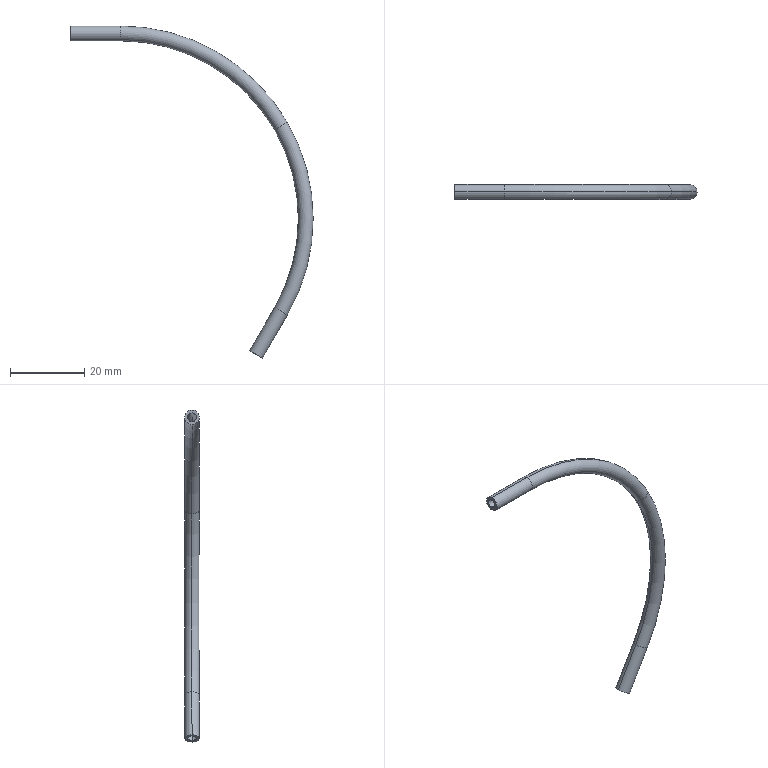Component | SolidWorks | WaterPipe1-2 | 1 solid | 18 faces | box 65.4 x 4 x 89.6 mm | volume 1058 mm3 | torus 8 | cylinder 8 | plane 2 | commonest cylinder face diameters 2.4 x4 4 x4
build123d program:
from build123d import *

# Parameters (mm, degrees)
SCAN_THIN_FEATURE1_PROFILE_R   = 2
SCAN_THIN_FEATURE1_PROFILE_R_2 = 1.2


with BuildPart() as part:
    # Scan-Thin Feature1: sweep along a path in Sketch1
    with BuildLine(Plane(origin=(0, 0, 0), x_dir=(1, 0, 0), z_dir=(0, 1, 0))) as scan_thin_feature1_path:
        Line((-50, 86.603), (-43.301, 75))
        ThreePointArc((-43.301, 75), (0, 50), (43.301, 75))
        Line((43.301, 75), (50, 86.603))
    # Scan-Thin Feature1 profile (on start of the path) → Scan-Thin Feature1 (sweep)
    with BuildSketch(Plane(origin=(-50, 0, -86.603), x_dir=(0.866, 0, -0.5), z_dir=(0.5, 0, 0.866))):
        Circle(SCAN_THIN_FEATURE1_PROFILE_R)
        Circle(SCAN_THIN_FEATURE1_PROFILE_R_2, mode=Mode.SUBTRACT)
    sweep(path=scan_thin_feature1_path.line)


solid = part.part

# Placed as in the assembly
solid = solid.moved(Location((104.985, 33.561, 224.066), (0, 60, 0)))
STEP:
#1=CARTESIAN_POINT('',(2.388,1.321,5.892));
#2=VERTEX_POINT('',#1);
#3=CARTESIAN_POINT('',(2.469,1.321,5.845));
#4=VERTEX_POINT('',#3);
#5=CARTESIAN_POINT('',(2.429,1.321,5.869));
#6=DIRECTION('',(-0.5,-0.,-0.866));
#7=DIRECTION('',(-0.866,0.,0.5));
#8=AXIS2_PLACEMENT_3D('',#5,#6,#7);
#9=CIRCLE('',#8,0.04724);
#10=EDGE_CURVE('',#2,#4,#9,.T.);
#11=ORIENTED_EDGE('',*,*,#10,.T.);
#12=CARTESIAN_POINT('',(2.469,1.321,7.861));
#13=VERTEX_POINT('',#12);
#14=CARTESIAN_POINT('',(0.7237,1.321,6.853));
#15=DIRECTION('',(0.,-1.,-0.));
#16=DIRECTION('',(1.,0.,0.));
#17=AXIS2_PLACEMENT_3D('',#14,#15,#16);
#18=CIRCLE('',#17,2.016);
#19=EDGE_CURVE('',#4,#13,#18,.T.);
#20=ORIENTED_EDGE('',*,*,#19,.T.);
#21=CARTESIAN_POINT('',(2.388,1.321,7.814));
#22=VERTEX_POINT('',#21);
#23=CARTESIAN_POINT('',(2.429,1.321,7.837));
#24=DIRECTION('',(0.5,0.,-0.866));
#25=DIRECTION('',(-0.866,0.,-0.5));
#26=AXIS2_PLACEMENT_3D('',#23,#24,#25);
#27=CIRCLE('',#26,0.04724);
#28=EDGE_CURVE('',#22,#13,#27,.T.);
#29=ORIENTED_EDGE('',*,*,#28,.F.);
#30=CARTESIAN_POINT('',(0.7237,1.321,6.853));
#31=DIRECTION('',(0.,-1.,-0.));
#32=DIRECTION('',(1.,0.,0.));
#33=AXIS2_PLACEMENT_3D('',#30,#31,#32);
#34=CIRCLE('',#33,1.921);
#35=EDGE_CURVE('',#2,#22,#34,.T.);
#36=ORIENTED_EDGE('',*,*,#35,.F.);
#37=EDGE_LOOP('',(#11,#20,#29,#36));
#38=FACE_OUTER_BOUND('',#37,.T.);
#39=CARTESIAN_POINT('',(0.7237,1.321,6.853));
#40=DIRECTION('',(0.,-1.,-0.));
#41=DIRECTION('',(0.866,0.,0.5));
#42=AXIS2_PLACEMENT_3D('',#39,#40,#41);
#43=TOROIDAL_SURFACE('',#42,1.969,0.04724);
#44=ADVANCED_FACE('',(#38),#43,.F.);
#45=CARTESIAN_POINT('',(2.497,1.321,7.877));
#46=VERTEX_POINT('',#45);
#47=CARTESIAN_POINT('',(2.36,1.321,7.798));
#48=VERTEX_POINT('',#47);
#49=CARTESIAN_POINT('',(2.429,1.321,7.837));
#50=DIRECTION('',(0.5,0.,-0.866));
#51=DIRECTION('',(-0.866,0.,-0.5));
#52=AXIS2_PLACEMENT_3D('',#49,#50,#51);
#53=CIRCLE('',#52,0.07874);
#54=EDGE_CURVE('',#46,#48,#53,.T.);
#55=ORIENTED_EDGE('',*,*,#54,.F.);
#56=CARTESIAN_POINT('',(0.7237,1.321,8.9));
#57=VERTEX_POINT('',#56);
#58=CARTESIAN_POINT('',(0.7237,1.321,6.853));
#59=DIRECTION('',(0.,-1.,-0.));
#60=DIRECTION('',(1.,0.,0.));
#61=AXIS2_PLACEMENT_3D('',#58,#59,#60);
#62=CIRCLE('',#61,2.047);
#63=EDGE_CURVE('',#46,#57,#62,.T.);
#64=ORIENTED_EDGE('',*,*,#63,.T.);
#65=CARTESIAN_POINT('',(0.7237,1.321,8.743));
#66=VERTEX_POINT('',#65);
#67=CARTESIAN_POINT('',(0.7237,1.321,8.822));
#68=DIRECTION('',(1.,0.,-0.));
#69=DIRECTION('',(0.,0.,1.));
#70=AXIS2_PLACEMENT_3D('',#67,#68,#69);
#71=CIRCLE('',#70,0.07874);
#72=EDGE_CURVE('',#57,#66,#71,.T.);
#73=ORIENTED_EDGE('',*,*,#72,.T.);
#74=CARTESIAN_POINT('',(0.7237,1.321,6.853));
#75=DIRECTION('',(0.,-1.,-0.));
#76=DIRECTION('',(1.,0.,0.));
#77=AXIS2_PLACEMENT_3D('',#74,#75,#76);
#78=CIRCLE('',#77,1.89);
#79=EDGE_CURVE('',#48,#66,#78,.T.);
#80=ORIENTED_EDGE('',*,*,#79,.F.);
#81=EDGE_LOOP('',(#55,#64,#73,#80));
#82=FACE_OUTER_BOUND('',#81,.T.);
#83=CARTESIAN_POINT('',(0.7237,1.321,6.853));
#84=DIRECTION('',(0.,-1.,-0.));
#85=DIRECTION('',(0.866,0.,0.5));
#86=AXIS2_PLACEMENT_3D('',#83,#84,#85);
#87=TOROIDAL_SURFACE('',#86,1.969,0.07874);
#88=ADVANCED_FACE('',(#82),#87,.T.);
#89=CARTESIAN_POINT('',(2.497,1.321,5.829));
#90=VERTEX_POINT('',#89);
#91=CARTESIAN_POINT('',(2.36,1.321,5.908));
#92=VERTEX_POINT('',#91);
#93=CARTESIAN_POINT('',(2.429,1.321,5.869));
#94=DIRECTION('',(-0.5,-0.,-0.866));
#95=DIRECTION('',(0.866,0.,-0.5));
#96=AXIS2_PLACEMENT_3D('',#93,#94,#95);
#97=CIRCLE('',#96,0.07874);
#98=EDGE_CURVE('',#90,#92,#97,.T.);
#99=ORIENTED_EDGE('',*,*,#98,.F.);
#100=CARTESIAN_POINT('',(0.7237,1.321,6.853));
#101=DIRECTION('',(0.,-1.,-0.));
#102=DIRECTION('',(1.,0.,0.));
#103=AXIS2_PLACEMENT_3D('',#100,#101,#102);
#104=CIRCLE('',#103,2.047);
#105=EDGE_CURVE('',#90,#46,#104,.T.);
#106=ORIENTED_EDGE('',*,*,#105,.T.);
#107=ORIENTED_EDGE('',*,*,#54,.T.);
#108=CARTESIAN_POINT('',(0.7237,1.321,6.853));
#109=DIRECTION('',(0.,-1.,-0.));
#110=DIRECTION('',(1.,0.,0.));
#111=AXIS2_PLACEMENT_3D('',#108,#109,#110);
#112=CIRCLE('',#111,1.89);
#113=EDGE_CURVE('',#92,#48,#112,.T.);
#114=ORIENTED_EDGE('',*,*,#113,.F.);
#115=EDGE_LOOP('',(#99,#106,#107,#114));
#116=FACE_OUTER_BOUND('',#115,.T.);
#117=CARTESIAN_POINT('',(0.7237,1.321,6.853));
#118=DIRECTION('',(0.,-1.,-0.));
#119=DIRECTION('',(0.866,0.,0.5));
#120=AXIS2_PLACEMENT_3D('',#117,#118,#119);
#121=TOROIDAL_SURFACE('',#120,1.969,0.07874);
#122=ADVANCED_FACE('',(#116),#121,.T.);
#123=ORIENTED_EDGE('',*,*,#28,.T.);
#124=CARTESIAN_POINT('',(0.7237,1.321,8.869));
#125=VERTEX_POINT('',#124);
#126=CARTESIAN_POINT('',(0.7237,1.321,6.853));
#127=DIRECTION('',(0.,-1.,-0.));
#128=DIRECTION('',(1.,0.,0.));
#129=AXIS2_PLACEMENT_3D('',#126,#127,#128);
#130=CIRCLE('',#129,2.016);
#131=EDGE_CURVE('',#13,#125,#130,.T.);
#132=ORIENTED_EDGE('',*,*,#131,.T.);
#133=CARTESIAN_POINT('',(0.7237,1.321,8.774));
#134=VERTEX_POINT('',#133);
#135=CARTESIAN_POINT('',(0.7237,1.321,8.822));
#136=DIRECTION('',(1.,0.,0.));
#137=DIRECTION('',(-0.,0.,1.));
#138=AXIS2_PLACEMENT_3D('',#135,#136,#137);
#139=CIRCLE('',#138,0.04724);
#140=EDGE_CURVE('',#134,#125,#139,.T.);
#141=ORIENTED_EDGE('',*,*,#140,.F.);
#142=CARTESIAN_POINT('',(0.7237,1.321,6.853));
#143=DIRECTION('',(0.,-1.,-0.));
#144=DIRECTION('',(1.,0.,0.));
#145=AXIS2_PLACEMENT_3D('',#142,#143,#144);
#146=CIRCLE('',#145,1.921);
#147=EDGE_CURVE('',#22,#134,#146,.T.);
#148=ORIENTED_EDGE('',*,*,#147,.F.);
#149=EDGE_LOOP('',(#123,#132,#141,#148));
#150=FACE_OUTER_BOUND('',#149,.T.);
#151=CARTESIAN_POINT('',(0.7237,1.321,6.853));
#152=DIRECTION('',(0.,-1.,-0.));
#153=DIRECTION('',(0.866,0.,0.5));
#154=AXIS2_PLACEMENT_3D('',#151,#152,#153);
#155=TOROIDAL_SURFACE('',#154,1.969,0.04724);
#156=ADVANCED_FACE('',(#150),#155,.F.);
#157=ORIENTED_EDGE('',*,*,#140,.T.);
#158=CARTESIAN_POINT('',(0.1963,1.321,8.869));
#159=VERTEX_POINT('',#158);
#160=CARTESIAN_POINT('',(0.7237,1.321,8.869));
#161=DIRECTION('',(-1.,-0.,0.));
#162=VECTOR('',#161,39.37);
#163=LINE('',#160,#162);
#164=EDGE_CURVE('',#125,#159,#163,.T.);
#165=ORIENTED_EDGE('',*,*,#164,.T.);
#166=CARTESIAN_POINT('',(0.1963,1.321,8.774));
#167=VERTEX_POINT('',#166);
#168=CARTESIAN_POINT('',(0.1963,1.321,8.822));
#169=DIRECTION('',(1.,0.,-0.));
#170=DIRECTION('',(0.,0.,1.));
#171=AXIS2_PLACEMENT_3D('',#168,#169,#170);
#172=CIRCLE('',#171,0.04724);
#173=EDGE_CURVE('',#167,#159,#172,.T.);
#174=ORIENTED_EDGE('',*,*,#173,.F.);
#175=CARTESIAN_POINT('',(0.7237,1.321,8.774));
#176=DIRECTION('',(-1.,-0.,0.));
#177=VECTOR('',#176,39.37);
#178=LINE('',#175,#177);
#179=EDGE_CURVE('',#134,#167,#178,.T.);
#180=ORIENTED_EDGE('',*,*,#179,.F.);
#181=EDGE_LOOP('',(#157,#165,#174,#180));
#182=FACE_OUTER_BOUND('',#181,.T.);
#183=CARTESIAN_POINT('',(0.7237,1.321,8.822));
#184=DIRECTION('',(-1.,-0.,0.));
#185=DIRECTION('',(0.,0.,-1.));
#186=AXIS2_PLACEMENT_3D('',#183,#184,#185);
#187=CYLINDRICAL_SURFACE('',#186,0.04724);
#188=ADVANCED_FACE('',(#182),#187,.F.);
#189=ORIENTED_EDGE('',*,*,#131,.F.);
#190=CARTESIAN_POINT('',(2.429,1.321,7.837));
#191=DIRECTION('',(0.5,0.,-0.866));
#192=DIRECTION('',(-0.866,0.,-0.5));
#193=AXIS2_PLACEMENT_3D('',#190,#191,#192);
#194=CIRCLE('',#193,0.04724);
#195=EDGE_CURVE('',#13,#22,#194,.T.);
#196=ORIENTED_EDGE('',*,*,#195,.T.);
#197=ORIENTED_EDGE('',*,*,#147,.T.);
#198=CARTESIAN_POINT('',(0.7237,1.321,8.822));
#199=DIRECTION('',(1.,0.,0.));
#200=DIRECTION('',(-0.,0.,1.));
#201=AXIS2_PLACEMENT_3D('',#198,#199,#200);
#202=CIRCLE('',#201,0.04724);
#203=EDGE_CURVE('',#125,#134,#202,.T.);
#204=ORIENTED_EDGE('',*,*,#203,.F.);
#205=EDGE_LOOP('',(#189,#196,#197,#204));
#206=FACE_OUTER_BOUND('',#205,.T.);
#207=CARTESIAN_POINT('',(0.7237,1.321,6.853));
#208=DIRECTION('',(0.,-1.,-0.));
#209=DIRECTION('',(0.866,0.,0.5));
#210=AXIS2_PLACEMENT_3D('',#207,#208,#209);
#211=TOROIDAL_SURFACE('',#210,1.969,0.04724);
#212=ADVANCED_FACE('',(#206),#211,.F.);
#213=CARTESIAN_POINT('',(2.124,1.321,5.436));
#214=VERTEX_POINT('',#213);
#215=CARTESIAN_POINT('',(2.206,1.321,5.388));
#216=VERTEX_POINT('',#215);
#217=CARTESIAN_POINT('',(2.165,1.321,5.412));
#218=DIRECTION('',(-0.5,-0.,-0.866));
#219=DIRECTION('',(0.866,0.,-0.5));
#220=AXIS2_PLACEMENT_3D('',#217,#218,#219);
#221=CIRCLE('',#220,0.04724);
#222=EDGE_CURVE('',#214,#216,#221,.T.);
#223=ORIENTED_EDGE('',*,*,#222,.T.);
#224=CARTESIAN_POINT('',(2.206,1.321,5.388));
#225=DIRECTION('',(0.5,0.,0.866));
#226=VECTOR('',#225,39.37);
#227=LINE('',#224,#226);
#228=EDGE_CURVE('',#216,#4,#227,.T.);
#229=ORIENTED_EDGE('',*,*,#228,.T.);
#230=ORIENTED_EDGE('',*,*,#10,.F.);
#231=CARTESIAN_POINT('',(2.124,1.321,5.436));
#232=DIRECTION('',(0.5,0.,0.866));
#233=VECTOR('',#232,39.37);
#234=LINE('',#231,#233);
#235=EDGE_CURVE('',#214,#2,#234,.T.);
#236=ORIENTED_EDGE('',*,*,#235,.F.);
#237=EDGE_LOOP('',(#223,#229,#230,#236));
#238=FACE_OUTER_BOUND('',#237,.T.);
#239=CARTESIAN_POINT('',(2.165,1.321,5.412));
#240=DIRECTION('',(0.5,0.,0.866));
#241=DIRECTION('',(-0.866,0.,0.5));
#242=AXIS2_PLACEMENT_3D('',#239,#240,#241);
#243=CYLINDRICAL_SURFACE('',#242,0.04724);
#244=ADVANCED_FACE('',(#238),#243,.F.);
#245=ORIENTED_EDGE('',*,*,#72,.F.);
#246=CARTESIAN_POINT('',(0.1963,1.321,8.9));
#247=VERTEX_POINT('',#246);
#248=CARTESIAN_POINT('',(0.7237,1.321,8.9));
#249=DIRECTION('',(-1.,-0.,0.));
#250=VECTOR('',#249,39.37);
#251=LINE('',#248,#250);
#252=EDGE_CURVE('',#57,#247,#251,.T.);
#253=ORIENTED_EDGE('',*,*,#252,.T.);
#254=CARTESIAN_POINT('',(0.1963,1.321,8.743));
#255=VERTEX_POINT('',#254);
#256=CARTESIAN_POINT('',(0.1963,1.321,8.822));
#257=DIRECTION('',(1.,0.,-0.));
#258=DIRECTION('',(0.,0.,1.));
#259=AXIS2_PLACEMENT_3D('',#256,#257,#258);
#260=CIRCLE('',#259,0.07874);
#261=EDGE_CURVE('',#247,#255,#260,.T.);
#262=ORIENTED_EDGE('',*,*,#261,.T.);
#263=CARTESIAN_POINT('',(0.7237,1.321,8.743));
#264=DIRECTION('',(-1.,-0.,0.));
#265=VECTOR('',#264,39.37);
#266=LINE('',#263,#265);
#267=EDGE_CURVE('',#66,#255,#266,.T.);
#268=ORIENTED_EDGE('',*,*,#267,.F.);
#269=EDGE_LOOP('',(#245,#253,#262,#268));
#270=FACE_OUTER_BOUND('',#269,.T.);
#271=CARTESIAN_POINT('',(0.7237,1.321,8.822));
#272=DIRECTION('',(-1.,-0.,0.));
#273=DIRECTION('',(0.,0.,-1.));
#274=AXIS2_PLACEMENT_3D('',#271,#272,#273);
#275=CYLINDRICAL_SURFACE('',#274,0.07874);
#276=ADVANCED_FACE('',(#270),#275,.T.);
#277=ORIENTED_EDGE('',*,*,#105,.F.);
#278=CARTESIAN_POINT('',(2.429,1.321,5.869));
#279=DIRECTION('',(-0.5,-0.,-0.866));
#280=DIRECTION('',(0.866,0.,-0.5));
#281=AXIS2_PLACEMENT_3D('',#278,#279,#280);
#282=CIRCLE('',#281,0.07874);
#283=EDGE_CURVE('',#92,#90,#282,.T.);
#284=ORIENTED_EDGE('',*,*,#283,.F.);
#285=ORIENTED_EDGE('',*,*,#113,.T.);
#286=CARTESIAN_POINT('',(2.429,1.321,7.837));
#287=DIRECTION('',(0.5,0.,-0.866));
#288=DIRECTION('',(-0.866,0.,-0.5));
#289=AXIS2_PLACEMENT_3D('',#286,#287,#288);
#290=CIRCLE('',#289,0.07874);
#291=EDGE_CURVE('',#48,#46,#290,.T.);
#292=ORIENTED_EDGE('',*,*,#291,.T.);
#293=EDGE_LOOP('',(#277,#284,#285,#292));
#294=FACE_OUTER_BOUND('',#293,.T.);
#295=CARTESIAN_POINT('',(0.7237,1.321,6.853));
#296=DIRECTION('',(0.,-1.,-0.));
#297=DIRECTION('',(0.866,0.,0.5));
#298=AXIS2_PLACEMENT_3D('',#295,#296,#297);
#299=TOROIDAL_SURFACE('',#298,1.969,0.07874);
#300=ADVANCED_FACE('',(#294),#299,.T.);
#301=CARTESIAN_POINT('',(2.233,1.321,5.373));
#302=VERTEX_POINT('',#301);
#303=CARTESIAN_POINT('',(2.097,1.321,5.451));
#304=VERTEX_POINT('',#303);
#305=CARTESIAN_POINT('',(2.165,1.321,5.412));
#306=DIRECTION('',(-0.5,-0.,-0.866));
#307=DIRECTION('',(0.866,0.,-0.5));
#308=AXIS2_PLACEMENT_3D('',#305,#306,#307);
#309=CIRCLE('',#308,0.07874);
#310=EDGE_CURVE('',#302,#304,#309,.T.);
#311=ORIENTED_EDGE('',*,*,#310,.F.);
#312=CARTESIAN_POINT('',(2.233,1.321,5.373));
#313=DIRECTION('',(0.5,0.,0.866));
#314=VECTOR('',#313,39.37);
#315=LINE('',#312,#314);
#316=EDGE_CURVE('',#302,#90,#315,.T.);
#317=ORIENTED_EDGE('',*,*,#316,.T.);
#318=ORIENTED_EDGE('',*,*,#98,.T.);
#319=CARTESIAN_POINT('',(2.097,1.321,5.451));
#320=DIRECTION('',(0.5,0.,0.866));
#321=VECTOR('',#320,39.37);
#322=LINE('',#319,#321);
#323=EDGE_CURVE('',#304,#92,#322,.T.);
#324=ORIENTED_EDGE('',*,*,#323,.F.);
#325=EDGE_LOOP('',(#311,#317,#318,#324));
#326=FACE_OUTER_BOUND('',#325,.T.);
#327=CARTESIAN_POINT('',(2.165,1.321,5.412));
#328=DIRECTION('',(0.5,0.,0.866));
#329=DIRECTION('',(-0.866,0.,0.5));
#330=AXIS2_PLACEMENT_3D('',#327,#328,#329);
#331=CYLINDRICAL_SURFACE('',#330,0.07874);
#332=ADVANCED_FACE('',(#326),#331,.T.);
#333=ORIENTED_EDGE('',*,*,#252,.F.);
#334=CARTESIAN_POINT('',(0.7237,1.321,8.822));
#335=DIRECTION('',(1.,0.,-0.));
#336=DIRECTION('',(0.,0.,1.));
#337=AXIS2_PLACEMENT_3D('',#334,#335,#336);
#338=CIRCLE('',#337,0.07874);
#339=EDGE_CURVE('',#66,#57,#338,.T.);
#340=ORIENTED_EDGE('',*,*,#339,.F.);
#341=ORIENTED_EDGE('',*,*,#267,.T.);
#342=CARTESIAN_POINT('',(0.1963,1.321,8.822));
#343=DIRECTION('',(1.,0.,-0.));
#344=DIRECTION('',(0.,0.,1.));
#345=AXIS2_PLACEMENT_3D('',#342,#343,#344);
#346=CIRCLE('',#345,0.07874);
#347=EDGE_CURVE('',#255,#247,#346,.T.);
#348=ORIENTED_EDGE('',*,*,#347,.T.);
#349=EDGE_LOOP('',(#333,#340,#341,#348));
#350=FACE_OUTER_BOUND('',#349,.T.);
#351=CARTESIAN_POINT('',(0.7237,1.321,8.822));
#352=DIRECTION('',(-1.,-0.,0.));
#353=DIRECTION('',(0.,0.,-1.));
#354=AXIS2_PLACEMENT_3D('',#351,#352,#353);
#355=CYLINDRICAL_SURFACE('',#354,0.07874);
#356=ADVANCED_FACE('',(#350),#355,.T.);
#357=ORIENTED_EDGE('',*,*,#63,.F.);
#358=ORIENTED_EDGE('',*,*,#291,.F.);
#359=ORIENTED_EDGE('',*,*,#79,.T.);
#360=ORIENTED_EDGE('',*,*,#339,.T.);
#361=EDGE_LOOP('',(#357,#358,#359,#360));
#362=FACE_OUTER_BOUND('',#361,.T.);
#363=CARTESIAN_POINT('',(0.7237,1.321,6.853));
#364=DIRECTION('',(0.,-1.,-0.));
#365=DIRECTION('',(0.866,0.,0.5));
#366=AXIS2_PLACEMENT_3D('',#363,#364,#365);
#367=TOROIDAL_SURFACE('',#366,1.969,0.07874);
#368=ADVANCED_FACE('',(#362),#367,.T.);
#369=ORIENTED_EDGE('',*,*,#316,.F.);
#370=CARTESIAN_POINT('',(2.165,1.321,5.412));
#371=DIRECTION('',(-0.5,-0.,-0.866));
#372=DIRECTION('',(0.866,0.,-0.5));
#373=AXIS2_PLACEMENT_3D('',#370,#371,#372);
#374=CIRCLE('',#373,0.07874);
#375=EDGE_CURVE('',#304,#302,#374,.T.);
#376=ORIENTED_EDGE('',*,*,#375,.F.);
#377=ORIENTED_EDGE('',*,*,#323,.T.);
#378=ORIENTED_EDGE('',*,*,#283,.T.);
#379=EDGE_LOOP('',(#369,#376,#377,#378));
#380=FACE_OUTER_BOUND('',#379,.T.);
#381=CARTESIAN_POINT('',(2.165,1.321,5.412));
#382=DIRECTION('',(0.5,0.,0.866));
#383=DIRECTION('',(-0.866,0.,0.5));
#384=AXIS2_PLACEMENT_3D('',#381,#382,#383);
#385=CYLINDRICAL_SURFACE('',#384,0.07874);
#386=ADVANCED_FACE('',(#380),#385,.T.);
#387=ORIENTED_EDGE('',*,*,#173,.T.);
#388=CARTESIAN_POINT('',(0.1963,1.321,8.822));
#389=DIRECTION('',(1.,0.,-0.));
#390=DIRECTION('',(0.,0.,1.));
#391=AXIS2_PLACEMENT_3D('',#388,#389,#390);
#392=CIRCLE('',#391,0.04724);
#393=EDGE_CURVE('',#159,#167,#392,.T.);
#394=ORIENTED_EDGE('',*,*,#393,.T.);
#395=EDGE_LOOP('',(#387,#394));
#396=FACE_BOUND('',#395,.T.);
#397=ORIENTED_EDGE('',*,*,#347,.F.);
#398=ORIENTED_EDGE('',*,*,#261,.F.);
#399=EDGE_LOOP('',(#397,#398));
#400=FACE_OUTER_BOUND('',#399,.T.);
#401=CARTESIAN_POINT('',(0.1963,1.321,8.822));
#402=DIRECTION('',(1.,0.,-0.));
#403=DIRECTION('',(0.,0.,1.));
#404=AXIS2_PLACEMENT_3D('',#401,#402,#403);
#405=PLANE('',#404);
#406=ADVANCED_FACE('',(#396,#400),#405,.F.);
#407=ORIENTED_EDGE('',*,*,#222,.F.);
#408=CARTESIAN_POINT('',(2.165,1.321,5.412));
#409=DIRECTION('',(-0.5,-0.,-0.866));
#410=DIRECTION('',(0.866,0.,-0.5));
#411=AXIS2_PLACEMENT_3D('',#408,#409,#410);
#412=CIRCLE('',#411,0.04724);
#413=EDGE_CURVE('',#216,#214,#412,.T.);
#414=ORIENTED_EDGE('',*,*,#413,.F.);
#415=EDGE_LOOP('',(#407,#414));
#416=FACE_BOUND('',#415,.T.);
#417=ORIENTED_EDGE('',*,*,#375,.T.);
#418=ORIENTED_EDGE('',*,*,#310,.T.);
#419=EDGE_LOOP('',(#417,#418));
#420=FACE_OUTER_BOUND('',#419,.T.);
#421=CARTESIAN_POINT('',(2.165,1.321,5.412));
#422=DIRECTION('',(-0.5,-0.,-0.866));
#423=DIRECTION('',(0.866,0.,-0.5));
#424=AXIS2_PLACEMENT_3D('',#421,#422,#423);
#425=PLANE('',#424);
#426=ADVANCED_FACE('',(#416,#420),#425,.T.);
#427=ORIENTED_EDGE('',*,*,#164,.F.);
#428=ORIENTED_EDGE('',*,*,#203,.T.);
#429=ORIENTED_EDGE('',*,*,#179,.T.);
#430=ORIENTED_EDGE('',*,*,#393,.F.);
#431=EDGE_LOOP('',(#427,#428,#429,#430));
#432=FACE_OUTER_BOUND('',#431,.T.);
#433=CARTESIAN_POINT('',(0.7237,1.321,8.822));
#434=DIRECTION('',(-1.,-0.,0.));
#435=DIRECTION('',(0.,0.,-1.));
#436=AXIS2_PLACEMENT_3D('',#433,#434,#435);
#437=CYLINDRICAL_SURFACE('',#436,0.04724);
#438=ADVANCED_FACE('',(#432),#437,.F.);
#439=ORIENTED_EDGE('',*,*,#19,.F.);
#440=CARTESIAN_POINT('',(2.429,1.321,5.869));
#441=DIRECTION('',(-0.5,-0.,-0.866));
#442=DIRECTION('',(-0.866,0.,0.5));
#443=AXIS2_PLACEMENT_3D('',#440,#441,#442);
#444=CIRCLE('',#443,0.04724);
#445=EDGE_CURVE('',#4,#2,#444,.T.);
#446=ORIENTED_EDGE('',*,*,#445,.T.);
#447=ORIENTED_EDGE('',*,*,#35,.T.);
#448=ORIENTED_EDGE('',*,*,#195,.F.);
#449=EDGE_LOOP('',(#439,#446,#447,#448));
#450=FACE_OUTER_BOUND('',#449,.T.);
#451=CARTESIAN_POINT('',(0.7237,1.321,6.853));
#452=DIRECTION('',(0.,-1.,-0.));
#453=DIRECTION('',(0.866,0.,0.5));
#454=AXIS2_PLACEMENT_3D('',#451,#452,#453);
#455=TOROIDAL_SURFACE('',#454,1.969,0.04724);
#456=ADVANCED_FACE('',(#450),#455,.F.);
#457=ORIENTED_EDGE('',*,*,#228,.F.);
#458=ORIENTED_EDGE('',*,*,#413,.T.);
#459=ORIENTED_EDGE('',*,*,#235,.T.);
#460=ORIENTED_EDGE('',*,*,#445,.F.);
#461=EDGE_LOOP('',(#457,#458,#459,#460));
#462=FACE_OUTER_BOUND('',#461,.T.);
#463=CARTESIAN_POINT('',(2.165,1.321,5.412));
#464=DIRECTION('',(0.5,0.,0.866));
#465=DIRECTION('',(-0.866,0.,0.5));
#466=AXIS2_PLACEMENT_3D('',#463,#464,#465);
#467=CYLINDRICAL_SURFACE('',#466,0.04724);
#468=ADVANCED_FACE('',(#462),#467,.F.);
#469=CLOSED_SHELL('',(#44,#88,#122,#156,#188,#212,#244,#276,#300,#332,#356,#368,#386,#406,#426,#438,#456,#468));
#470=MANIFOLD_SOLID_BREP('',#469);
#471=CARTESIAN_POINT('',(0.,0.,0.));
#472=DIRECTION('',(0.,0.,1.));
#473=DIRECTION('',(1.,0.,0.));
#474=AXIS2_PLACEMENT_3D('',#471,#472,#473);
#475=(LENGTH_UNIT()NAMED_UNIT(*)SI_UNIT($,.METRE.));
#476=LENGTH_MEASURE_WITH_UNIT(LENGTH_MEASURE(0.0254),#475);
#477=DIMENSIONAL_EXPONENTS(1.,0.,0.,0.,0.,0.,0.);
#478=(CONVERSION_BASED_UNIT('',#476)LENGTH_UNIT()NAMED_UNIT(#477));
#479=UNCERTAINTY_MEASURE_WITH_UNIT(LENGTH_MEASURE(0.00001),#478,'','');
#480=(NAMED_UNIT(*)PLANE_ANGLE_UNIT()SI_UNIT($,.RADIAN.));
#481=(NAMED_UNIT(*)SI_UNIT($,.STERADIAN.)SOLID_ANGLE_UNIT());
#482=(GEOMETRIC_REPRESENTATION_CONTEXT(3)GLOBAL_UNCERTAINTY_ASSIGNED_CONTEXT((#479))GLOBAL_UNIT_ASSIGNED_CONTEXT((#478,#480,#481))REPRESENTATION_CONTEXT('',''));
#483=ADVANCED_BREP_SHAPE_REPRESENTATION('',(#470,#474),#482);
#484=COLOUR_RGB('',0.7922,0.8196,0.9333);
#485=FILL_AREA_STYLE_COLOUR('',#484);
#486=FILL_AREA_STYLE('',(#485));
#487=SURFACE_STYLE_FILL_AREA(#486);
#488=SURFACE_SIDE_STYLE('',(#487));
#489=SURFACE_STYLE_USAGE(.BOTH.,#488);
#490=PRESENTATION_STYLE_ASSIGNMENT((#489));
#491=STYLED_ITEM('',(#490),#470);
#492=PRESENTATION_LAYER_ASSIGNMENT('','',(#491));
#493=(LENGTH_UNIT()NAMED_UNIT(*)SI_UNIT($,.METRE.));
#494=LENGTH_MEASURE_WITH_UNIT(LENGTH_MEASURE(0.0254),#493);
#495=DIMENSIONAL_EXPONENTS(1.,0.,0.,0.,0.,0.,0.);
#496=(CONVERSION_BASED_UNIT('',#494)LENGTH_UNIT()NAMED_UNIT(#495));
#497=UNCERTAINTY_MEASURE_WITH_UNIT(LENGTH_MEASURE(0.00001),#496,'','');
#498=(NAMED_UNIT(*)PLANE_ANGLE_UNIT()SI_UNIT($,.RADIAN.));
#499=(NAMED_UNIT(*)SI_UNIT($,.STERADIAN.)SOLID_ANGLE_UNIT());
#500=(GEOMETRIC_REPRESENTATION_CONTEXT(3)GLOBAL_UNCERTAINTY_ASSIGNED_CONTEXT((#497))GLOBAL_UNIT_ASSIGNED_CONTEXT((#496,#498,#499))REPRESENTATION_CONTEXT('',''));
#501=MECHANICAL_DESIGN_GEOMETRIC_PRESENTATION_REPRESENTATION('',(#491),#500);